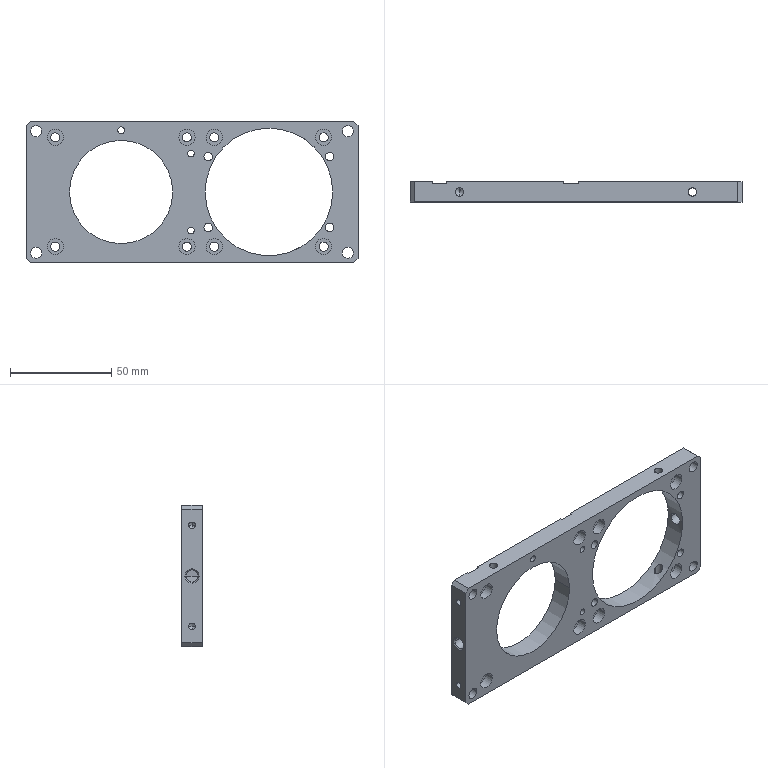CAM job | Mastercam | mm | 17 operations | part box 164 x 10 x 70
1. Facing | 20 - 63 平铣刀
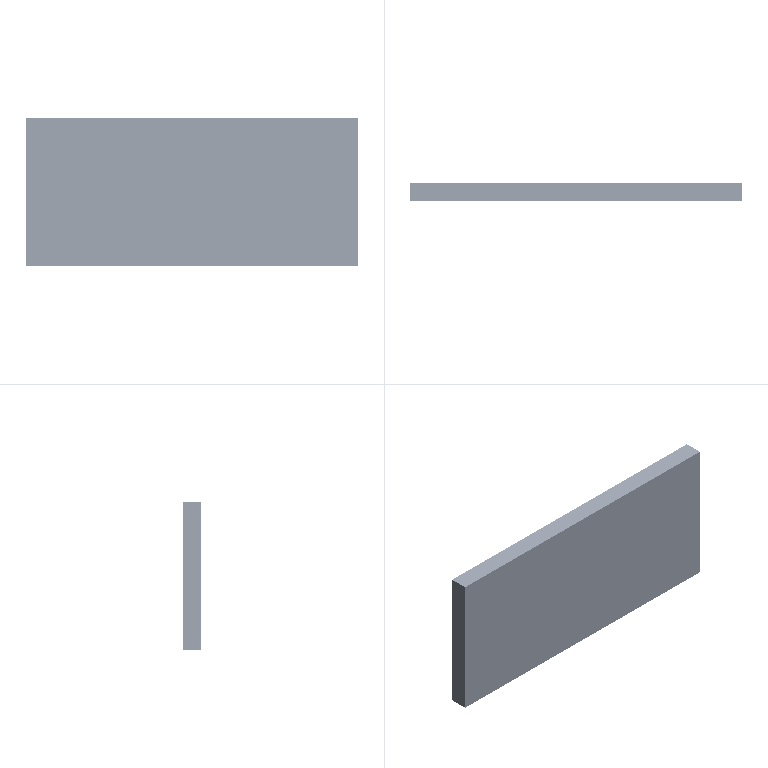2. Contour (Ramp) | 10 - 10 平铣刀
3. 2D High Speed (2D Dynamic Mill) | 10 - 10 平铣刀
4. Contour (2D) | 10 - 10 平铣刀
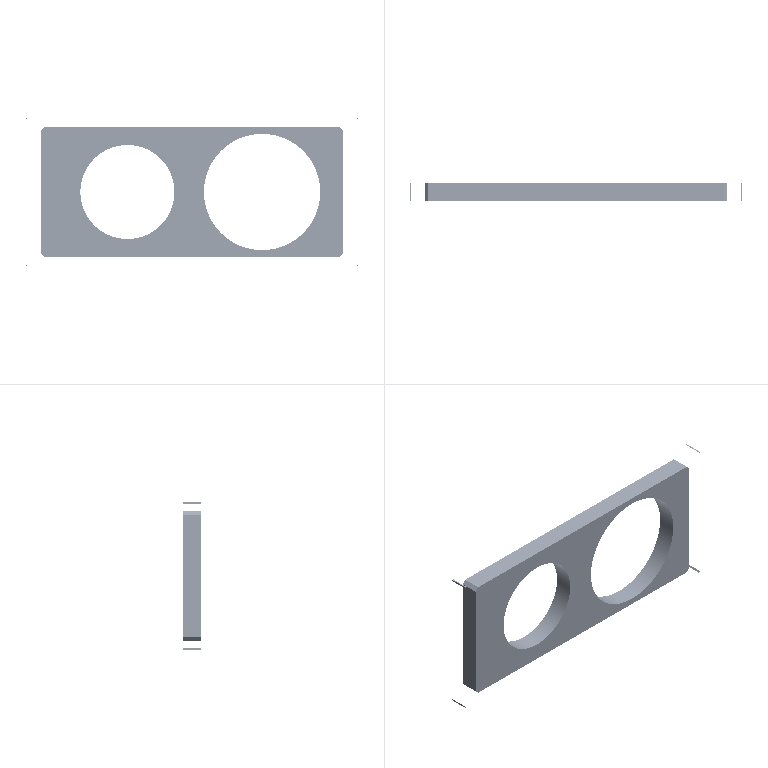5. Contour (Ramp) | 6 - 6 平铣刀
6. Contour (Ramp) | 6 - 6 平铣刀
7. Contour (2D) | 6 - 6 平铣刀
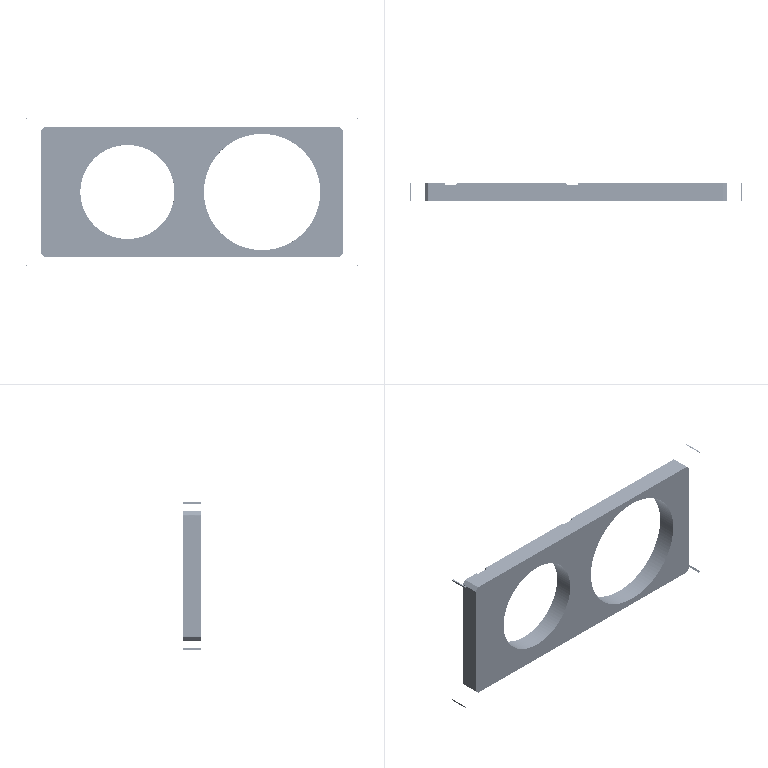8. Contour (2D) | 6 - 6 平铣刀
9. Contour (2D chamfer) | 7 - 4 倒角刀
10. Contour (2D chamfer) | 7 - 4 倒角刀
11. Facing | 20 - 63 平铣刀
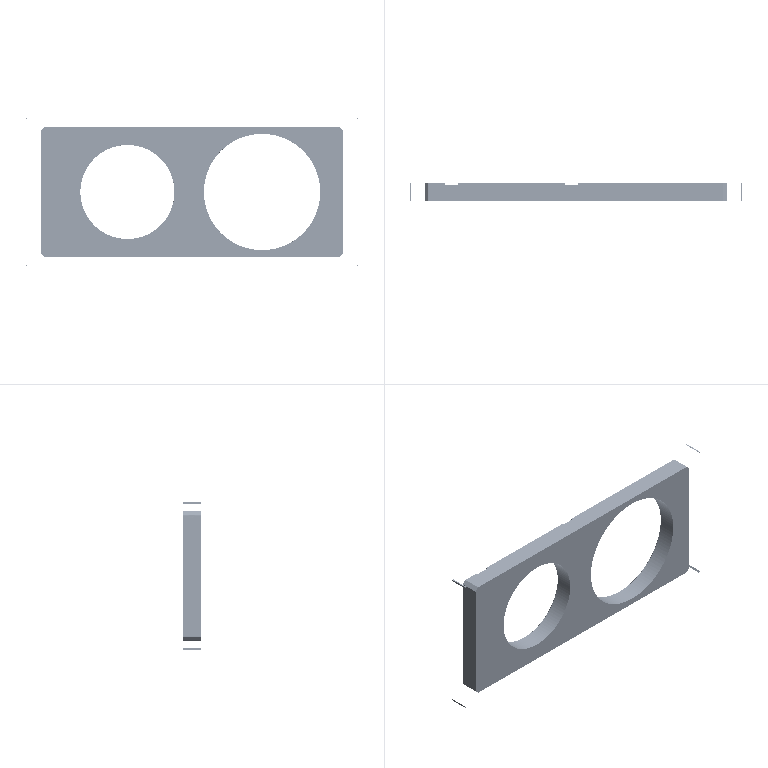12. Contour (Ramp) | 6 - 6 平铣刀
13. Contour (2D chamfer) | 7 - 4 倒角刀
14. Contour (2D chamfer) | 7 - 4 倒角刀
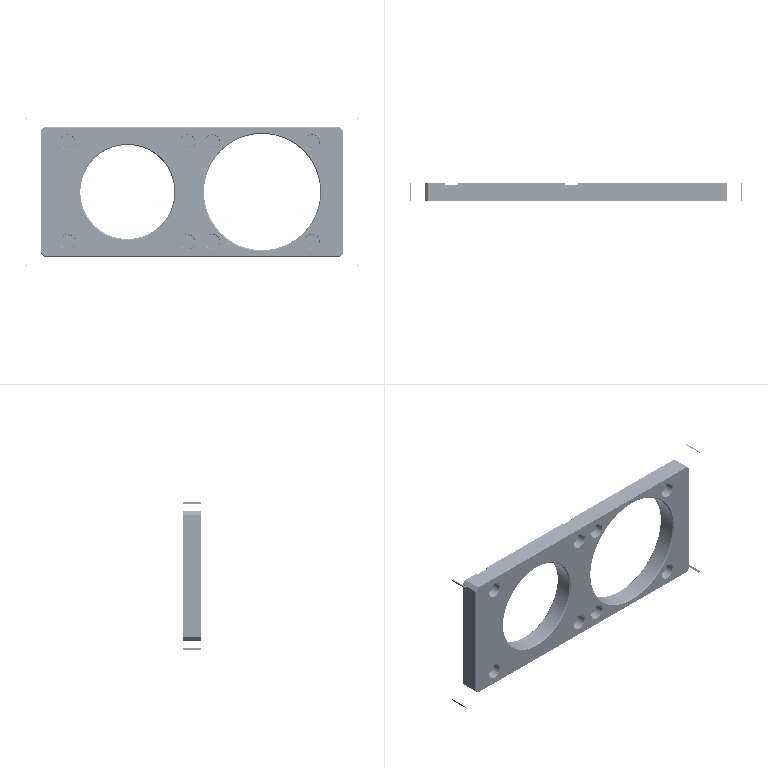15. Drill/Counterbore | 7 - 4 倒角刀
16. Drill/Counterbore | 7 - 4 倒角刀
17. Drill/Counterbore | 7 - 4 倒角刀